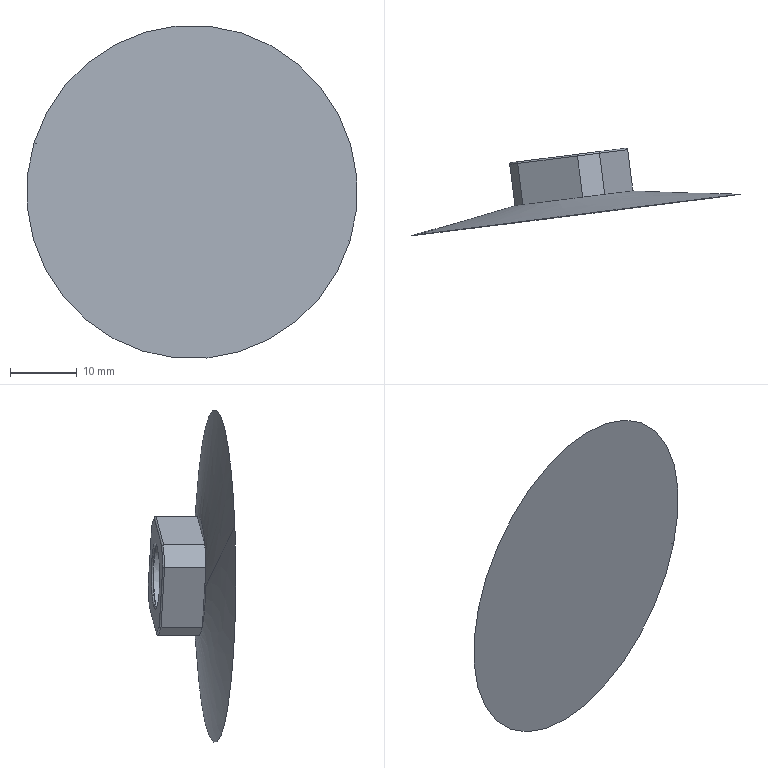Component | SolidWorks | SuctionCup-1 | 1 solid | 35 faces | box 49.61 x 13.13 x 50 mm | volume 3362 mm3 | plane 19 | cylinder 8 | torus 4 | spline 2 | sphere 2 | commonest cylinder face diameters 0.5 x8
STEP:
#1=COLOUR_RGB('',0.7922,0.8196,0.9333);
#2=FILL_AREA_STYLE_COLOUR('',#1);
#3=FILL_AREA_STYLE('',(#2));
#4=SURFACE_STYLE_FILL_AREA(#3);
#5=SURFACE_SIDE_STYLE('',(#4));
#6=SURFACE_STYLE_USAGE(.BOTH.,#5);
#7=PRESENTATION_STYLE_ASSIGNMENT((#6));
#8=CARTESIAN_POINT('',(20.728,-12.767,5.415));
#9=VERTEX_POINT('',#8);
#10=CARTESIAN_POINT('',(20.728,-12.77,5.415));
#11=VERTEX_POINT('',#10);
#12=CARTESIAN_POINT('',(20.724,-12.767,5.424));
#13=DIRECTION('',(-0.8974,-0.113,-0.4265));
#14=DIRECTION('',(-0.4293,0.,0.9032));
#15=AXIS2_PLACEMENT_3D('',#12,#13,#14);
#16=CIRCLE('',#15,0.009843);
#17=EDGE_CURVE('',#9,#11,#16,.T.);
#18=ORIENTED_EDGE('',*,*,#17,.F.);
#19=CARTESIAN_POINT('',(20.887,-12.747,5.074));
#20=VERTEX_POINT('',#19);
#21=CARTESIAN_POINT('',(20.808,-12.757,5.245));
#22=DIRECTION('',(-0.1249,0.9922,-0.));
#23=DIRECTION('',(-0.9922,-0.1249,0.));
#24=AXIS2_PLACEMENT_3D('',#21,#22,#23);
#25=CIRCLE('',#24,0.1882);
#26=EDGE_CURVE('',#9,#20,#25,.T.);
#27=ORIENTED_EDGE('',*,*,#26,.T.);
#28=CARTESIAN_POINT('',(20.888,-12.75,5.074));
#29=VERTEX_POINT('',#28);
#30=CARTESIAN_POINT('',(20.891,-12.746,5.065));
#31=DIRECTION('',(0.8974,0.113,0.4265));
#32=DIRECTION('',(0.4293,0.,-0.9032));
#33=AXIS2_PLACEMENT_3D('',#30,#31,#32);
#34=CIRCLE('',#33,0.009843);
#35=EDGE_CURVE('',#20,#29,#34,.T.);
#36=ORIENTED_EDGE('',*,*,#35,.T.);
#37=CARTESIAN_POINT('',(20.808,-12.76,5.245));
#38=DIRECTION('',(-0.1249,0.9922,-0.));
#39=DIRECTION('',(-0.4232,-0.05327,0.9045));
#40=AXIS2_PLACEMENT_3D('',#37,#38,#39);
#41=CIRCLE('',#40,0.1886);
#42=EDGE_CURVE('',#11,#29,#41,.T.);
#43=ORIENTED_EDGE('',*,*,#42,.F.);
#44=EDGE_LOOP('',(#18,#27,#36,#43));
#45=FACE_OUTER_BOUND('',#44,.T.);
#46=CARTESIAN_POINT('',(20.808,-12.757,5.245));
#47=DIRECTION('',(-0.1249,0.9922,-0.));
#48=DIRECTION('',(0.4232,0.05327,-0.9045));
#49=AXIS2_PLACEMENT_3D('',#46,#47,#48);
#50=TOROIDAL_SURFACE('',#49,0.1981,0.009843);
#51=ADVANCED_FACE('',(#45),#50,.T.);
#52=ORIENTED_EDGE('',*,*,#35,.F.);
#53=CARTESIAN_POINT('',(20.808,-12.757,5.245));
#54=DIRECTION('',(-0.1249,0.9922,-0.));
#55=DIRECTION('',(-0.9922,-0.1249,0.));
#56=AXIS2_PLACEMENT_3D('',#53,#54,#55);
#57=CIRCLE('',#56,0.1882);
#58=EDGE_CURVE('',#20,#9,#57,.T.);
#59=ORIENTED_EDGE('',*,*,#58,.T.);
#60=ORIENTED_EDGE('',*,*,#17,.T.);
#61=CARTESIAN_POINT('',(20.808,-12.76,5.245));
#62=DIRECTION('',(-0.1249,0.9922,-0.));
#63=DIRECTION('',(-0.4232,-0.05327,0.9045));
#64=AXIS2_PLACEMENT_3D('',#61,#62,#63);
#65=CIRCLE('',#64,0.1886);
#66=EDGE_CURVE('',#29,#11,#65,.T.);
#67=ORIENTED_EDGE('',*,*,#66,.F.);
#68=EDGE_LOOP('',(#52,#59,#60,#67));
#69=FACE_OUTER_BOUND('',#68,.T.);
#70=CARTESIAN_POINT('',(20.808,-12.757,5.245));
#71=DIRECTION('',(-0.1249,0.9922,-0.));
#72=DIRECTION('',(0.4232,0.05327,-0.9045));
#73=AXIS2_PLACEMENT_3D('',#70,#71,#72);
#74=TOROIDAL_SURFACE('',#73,0.1981,0.009843);
#75=ADVANCED_FACE('',(#69),#74,.T.);
#76=CARTESIAN_POINT('',(21.187,-12.957,5.192));
#77=VERTEX_POINT('',#76);
#78=CARTESIAN_POINT('',(21.185,-12.957,5.304));
#79=VERTEX_POINT('',#78);
#80=CARTESIAN_POINT('',(20.838,-13.001,5.245));
#81=DIRECTION('',(0.1249,-0.9922,0.));
#82=DIRECTION('',(-0.4232,-0.05327,0.9045));
#83=AXIS2_PLACEMENT_3D('',#80,#81,#82);
#84=CIRCLE('',#83,0.3549);
#85=EDGE_CURVE('',#77,#79,#84,.T.);
#86=ORIENTED_EDGE('',*,*,#85,.T.);
#87=CARTESIAN_POINT('',(21.783,-12.981,4.952));
#88=VERTEX_POINT('',#87);
#89=CARTESIAN_POINT('',(21.185,-12.957,5.304));
#90=CARTESIAN_POINT('',(21.783,-12.981,4.952));
#91=B_SPLINE_CURVE_WITH_KNOTS('',1,(#89,#90),.UNSPECIFIED.,.F.,.F.,(2,2),(0.,1.),.UNSPECIFIED.);
#92=EDGE_CURVE('',#79,#88,#91,.T.);
#93=ORIENTED_EDGE('',*,*,#92,.T.);
#94=CARTESIAN_POINT('',(19.918,-13.216,5.537));
#95=VERTEX_POINT('',#94);
#96=CARTESIAN_POINT('',(20.851,-13.099,5.245));
#97=DIRECTION('',(0.1249,-0.9922,0.));
#98=DIRECTION('',(-0.4232,-0.05327,0.9045));
#99=AXIS2_PLACEMENT_3D('',#96,#97,#98);
#100=CIRCLE('',#99,0.9843);
#101=EDGE_CURVE('',#95,#88,#100,.T.);
#102=ORIENTED_EDGE('',*,*,#101,.F.);
#103=CARTESIAN_POINT('',(20.491,-13.045,5.185));
#104=VERTEX_POINT('',#103);
#105=CARTESIAN_POINT('',(20.491,-13.045,5.185));
#106=CARTESIAN_POINT('',(19.918,-13.216,5.537));
#107=B_SPLINE_CURVE_WITH_KNOTS('',1,(#105,#106),.UNSPECIFIED.,.F.,.F.,(2,2),(0.,1.),.UNSPECIFIED.);
#108=EDGE_CURVE('',#104,#95,#107,.T.);
#109=ORIENTED_EDGE('',*,*,#108,.F.);
#110=CARTESIAN_POINT('',(20.657,-13.024,4.941));
#111=VERTEX_POINT('',#110);
#112=CARTESIAN_POINT('',(20.838,-13.001,5.245));
#113=DIRECTION('',(0.1249,-0.9922,0.));
#114=DIRECTION('',(-0.4232,-0.05327,0.9045));
#115=AXIS2_PLACEMENT_3D('',#112,#113,#114);
#116=CIRCLE('',#115,0.3549);
#117=EDGE_CURVE('',#104,#111,#116,.T.);
#118=ORIENTED_EDGE('',*,*,#117,.T.);
#119=CARTESIAN_POINT('',(20.787,-13.007,4.894));
#120=VERTEX_POINT('',#119);
#121=CARTESIAN_POINT('',(20.838,-13.001,5.245));
#122=DIRECTION('',(0.1249,-0.9922,0.));
#123=DIRECTION('',(-0.4232,-0.05327,0.9045));
#124=AXIS2_PLACEMENT_3D('',#121,#122,#123);
#125=CIRCLE('',#124,0.3549);
#126=EDGE_CURVE('',#111,#120,#125,.T.);
#127=ORIENTED_EDGE('',*,*,#126,.T.);
#128=CARTESIAN_POINT('',(21.14,-12.963,5.061));
#129=VERTEX_POINT('',#128);
#130=CARTESIAN_POINT('',(20.838,-13.001,5.245));
#131=DIRECTION('',(0.1249,-0.9922,0.));
#132=DIRECTION('',(-0.4232,-0.05327,0.9045));
#133=AXIS2_PLACEMENT_3D('',#130,#131,#132);
#134=CIRCLE('',#133,0.3549);
#135=EDGE_CURVE('',#120,#129,#134,.T.);
#136=ORIENTED_EDGE('',*,*,#135,.T.);
#137=CARTESIAN_POINT('',(20.838,-13.001,5.245));
#138=DIRECTION('',(0.1249,-0.9922,0.));
#139=DIRECTION('',(-0.4232,-0.05327,0.9045));
#140=AXIS2_PLACEMENT_3D('',#137,#138,#139);
#141=CIRCLE('',#140,0.3549);
#142=EDGE_CURVE('',#129,#77,#141,.T.);
#143=ORIENTED_EDGE('',*,*,#142,.T.);
#144=EDGE_LOOP('',(#86,#93,#102,#109,#118,#127,#136,#143));
#145=FACE_OUTER_BOUND('',#144,.T.);
#146=CARTESIAN_POINT('',(20.491,-13.045,5.185));
#147=CARTESIAN_POINT('',(19.918,-13.216,5.537));
#148=CARTESIAN_POINT('',(20.609,-13.03,4.485));
#149=CARTESIAN_POINT('',(19.337,-13.289,3.658));
#150=CARTESIAN_POINT('',(21.303,-12.942,4.604));
#151=CARTESIAN_POINT('',(21.202,-13.054,3.072));
#152=CARTESIAN_POINT('',(21.185,-12.957,5.304));
#153=CARTESIAN_POINT('',(21.783,-12.981,4.952));
#154=CARTESIAN_POINT('',(21.068,-12.972,6.004));
#155=CARTESIAN_POINT('',(22.364,-12.908,6.831));
#156=CARTESIAN_POINT('',(20.373,-13.059,5.885));
#157=CARTESIAN_POINT('',(20.499,-13.143,7.417));
#158=CARTESIAN_POINT('',(20.491,-13.045,5.185));
#159=CARTESIAN_POINT('',(19.918,-13.216,5.537));
#160=(BOUNDED_SURFACE()B_SPLINE_SURFACE(3,1,((#146,#147),(#148,#149),(#150,#151),(#152,#153),(#154,#155),(#156,#157),(#158,#159)),.UNSPECIFIED.,.T.,.F.,.F.)B_SPLINE_SURFACE_WITH_KNOTS((4,3,4),(2,2),(0.,0.5,1.),(0.,1.),.UNSPECIFIED.)GEOMETRIC_REPRESENTATION_ITEM()RATIONAL_B_SPLINE_SURFACE(((1.,1.),(0.3333,0.3333),(0.3333,0.3333),(1.,1.),(0.3333,0.3333),(0.3333,0.3333),(1.,1.)))REPRESENTATION_ITEM('')SURFACE());
#161=ADVANCED_FACE('',(#145),#160,.T.);
#162=ORIENTED_EDGE('',*,*,#58,.F.);
#163=CARTESIAN_POINT('',(20.89,-12.737,5.065));
#164=VERTEX_POINT('',#163);
#165=CARTESIAN_POINT('',(20.891,-12.746,5.065));
#166=DIRECTION('',(0.8974,0.113,0.4265));
#167=DIRECTION('',(0.4293,0.,-0.9032));
#168=AXIS2_PLACEMENT_3D('',#165,#166,#167);
#169=CIRCLE('',#168,0.009843);
#170=EDGE_CURVE('',#164,#20,#169,.T.);
#171=ORIENTED_EDGE('',*,*,#170,.F.);
#172=CARTESIAN_POINT('',(20.722,-12.758,5.424));
#173=VERTEX_POINT('',#172);
#174=CARTESIAN_POINT('',(20.806,-12.747,5.245));
#175=DIRECTION('',(0.1249,-0.9922,0.));
#176=DIRECTION('',(0.4232,0.05327,-0.9045));
#177=AXIS2_PLACEMENT_3D('',#174,#175,#176);
#178=CIRCLE('',#177,0.1981);
#179=EDGE_CURVE('',#173,#164,#178,.T.);
#180=ORIENTED_EDGE('',*,*,#179,.F.);
#181=CARTESIAN_POINT('',(20.724,-12.767,5.424));
#182=DIRECTION('',(-0.8974,-0.113,-0.4265));
#183=DIRECTION('',(-0.4293,0.,0.9032));
#184=AXIS2_PLACEMENT_3D('',#181,#182,#183);
#185=CIRCLE('',#184,0.009843);
#186=EDGE_CURVE('',#173,#9,#185,.T.);
#187=ORIENTED_EDGE('',*,*,#186,.T.);
#188=EDGE_LOOP('',(#162,#171,#180,#187));
#189=FACE_OUTER_BOUND('',#188,.T.);
#190=CARTESIAN_POINT('',(20.808,-12.757,5.245));
#191=DIRECTION('',(-0.1249,0.9922,-0.));
#192=DIRECTION('',(0.4232,0.05327,-0.9045));
#193=AXIS2_PLACEMENT_3D('',#190,#191,#192);
#194=TOROIDAL_SURFACE('',#193,0.1981,0.009843);
#195=ADVANCED_FACE('',(#189),#194,.T.);
#196=CARTESIAN_POINT('',(20.864,-12.998,5.189));
#197=VERTEX_POINT('',#196);
#198=CARTESIAN_POINT('',(20.812,-13.004,5.3));
#199=VERTEX_POINT('',#198);
#200=CARTESIAN_POINT('',(20.838,-13.001,5.245));
#201=DIRECTION('',(-0.1249,0.9922,-0.));
#202=DIRECTION('',(0.4232,0.05327,-0.9045));
#203=AXIS2_PLACEMENT_3D('',#200,#201,#202);
#204=CIRCLE('',#203,0.06147);
#205=EDGE_CURVE('',#197,#199,#204,.T.);
#206=ORIENTED_EDGE('',*,*,#205,.F.);
#207=CARTESIAN_POINT('',(20.815,-12.815,5.245));
#208=DIRECTION('',(0.8974,0.113,0.4265));
#209=DIRECTION('',(0.4293,0.,-0.9032));
#210=AXIS2_PLACEMENT_3D('',#207,#208,#209);
#211=CIRCLE('',#210,0.1969);
#212=EDGE_CURVE('',#197,#29,#211,.T.);
#213=ORIENTED_EDGE('',*,*,#212,.T.);
#214=ORIENTED_EDGE('',*,*,#66,.T.);
#215=CARTESIAN_POINT('',(20.815,-12.815,5.245));
#216=DIRECTION('',(-0.8974,-0.113,-0.4265));
#217=DIRECTION('',(-0.4293,0.,0.9032));
#218=AXIS2_PLACEMENT_3D('',#215,#216,#217);
#219=CIRCLE('',#218,0.1969);
#220=EDGE_CURVE('',#199,#11,#219,.T.);
#221=ORIENTED_EDGE('',*,*,#220,.F.);
#222=EDGE_LOOP('',(#206,#213,#214,#221));
#223=FACE_OUTER_BOUND('',#222,.T.);
#224=CARTESIAN_POINT('',(20.815,-12.815,5.245));
#225=DIRECTION('',(0.8974,0.113,0.4265));
#226=DIRECTION('',(-0.4232,-0.05327,0.9045));
#227=AXIS2_PLACEMENT_3D('',#224,#225,#226);
#228=SPHERICAL_SURFACE('',#227,0.1969);
#229=ADVANCED_FACE('',(#223),#228,.F.);
#230=CARTESIAN_POINT('',(20.89,-12.994,5.596));
#231=VERTEX_POINT('',#230);
#232=CARTESIAN_POINT('',(20.859,-12.75,5.596));
#233=VERTEX_POINT('',#232);
#234=CARTESIAN_POINT('',(20.89,-12.994,5.596));
#235=DIRECTION('',(-0.1249,0.9922,-0.));
#236=VECTOR('',#235,39.37);
#237=LINE('',#234,#236);
#238=EDGE_CURVE('',#231,#233,#237,.T.);
#239=ORIENTED_EDGE('',*,*,#238,.T.);
#240=CARTESIAN_POINT('',(20.506,-12.795,5.428));
#241=VERTEX_POINT('',#240);
#242=CARTESIAN_POINT('',(20.506,-12.795,5.428));
#243=DIRECTION('',(-0.8974,-0.113,-0.4265));
#244=VECTOR('',#243,39.37);
#245=LINE('',#242,#244);
#246=EDGE_CURVE('',#233,#241,#245,.T.);
#247=ORIENTED_EDGE('',*,*,#246,.T.);
#248=CARTESIAN_POINT('',(20.537,-13.039,5.428));
#249=VERTEX_POINT('',#248);
#250=CARTESIAN_POINT('',(20.537,-13.039,5.428));
#251=DIRECTION('',(0.1249,-0.9922,0.));
#252=VECTOR('',#251,39.37);
#253=LINE('',#250,#252);
#254=EDGE_CURVE('',#241,#249,#253,.T.);
#255=ORIENTED_EDGE('',*,*,#254,.T.);
#256=CARTESIAN_POINT('',(20.978,-12.983,5.638));
#257=DIRECTION('',(-0.8974,-0.113,-0.4265));
#258=VECTOR('',#257,39.37);
#259=LINE('',#256,#258);
#260=EDGE_CURVE('',#231,#249,#259,.T.);
#261=ORIENTED_EDGE('',*,*,#260,.F.);
#262=EDGE_LOOP('',(#239,#247,#255,#261));
#263=FACE_OUTER_BOUND('',#262,.T.);
#264=CARTESIAN_POINT('',(20.978,-12.983,5.638));
#265=DIRECTION('',(0.4232,0.05327,-0.9045));
#266=DIRECTION('',(0.1249,-0.9922,0.));
#267=AXIS2_PLACEMENT_3D('',#264,#265,#266);
#268=PLANE('',#267);
#269=ADVANCED_FACE('',(#263),#268,.F.);
#270=CARTESIAN_POINT('',(20.49,-13.045,5.297));
#271=VERTEX_POINT('',#270);
#272=CARTESIAN_POINT('',(20.459,-12.801,5.297));
#273=VERTEX_POINT('',#272);
#274=CARTESIAN_POINT('',(20.49,-13.045,5.297));
#275=DIRECTION('',(-0.1249,0.9922,-0.));
#276=VECTOR('',#275,39.37);
#277=LINE('',#274,#276);
#278=EDGE_CURVE('',#271,#273,#277,.T.);
#279=ORIENTED_EDGE('',*,*,#278,.T.);
#280=CARTESIAN_POINT('',(20.626,-12.78,4.941));
#281=VERTEX_POINT('',#280);
#282=CARTESIAN_POINT('',(20.626,-12.78,4.941));
#283=DIRECTION('',(0.4232,0.05327,-0.9045));
#284=VECTOR('',#283,39.37);
#285=LINE('',#282,#284);
#286=EDGE_CURVE('',#273,#281,#285,.T.);
#287=ORIENTED_EDGE('',*,*,#286,.T.);
#288=CARTESIAN_POINT('',(20.657,-13.024,4.941));
#289=DIRECTION('',(0.1249,-0.9922,0.));
#290=VECTOR('',#289,39.37);
#291=LINE('',#288,#290);
#292=EDGE_CURVE('',#281,#111,#291,.T.);
#293=ORIENTED_EDGE('',*,*,#292,.T.);
#294=CARTESIAN_POINT('',(20.698,-13.019,4.852));
#295=DIRECTION('',(0.4232,0.05327,-0.9045));
#296=VECTOR('',#295,39.37);
#297=LINE('',#294,#296);
#298=EDGE_CURVE('',#271,#111,#297,.T.);
#299=ORIENTED_EDGE('',*,*,#298,.F.);
#300=EDGE_LOOP('',(#279,#287,#293,#299));
#301=FACE_OUTER_BOUND('',#300,.T.);
#302=CARTESIAN_POINT('',(20.698,-13.019,4.852));
#303=DIRECTION('',(0.8974,0.113,0.4265));
#304=DIRECTION('',(-0.1249,0.9922,-0.));
#305=AXIS2_PLACEMENT_3D('',#302,#303,#304);
#306=PLANE('',#305);
#307=ADVANCED_FACE('',(#301),#306,.F.);
#308=CARTESIAN_POINT('',(20.756,-12.763,4.894));
#309=VERTEX_POINT('',#308);
#310=CARTESIAN_POINT('',(20.787,-13.007,4.894));
#311=DIRECTION('',(-0.1249,0.9922,-0.));
#312=VECTOR('',#311,39.37);
#313=LINE('',#310,#312);
#314=EDGE_CURVE('',#120,#309,#313,.T.);
#315=ORIENTED_EDGE('',*,*,#314,.T.);
#316=CARTESIAN_POINT('',(21.109,-12.719,5.061));
#317=VERTEX_POINT('',#316);
#318=CARTESIAN_POINT('',(21.109,-12.719,5.061));
#319=DIRECTION('',(0.8974,0.113,0.4265));
#320=VECTOR('',#319,39.37);
#321=LINE('',#318,#320);
#322=EDGE_CURVE('',#309,#317,#321,.T.);
#323=ORIENTED_EDGE('',*,*,#322,.T.);
#324=CARTESIAN_POINT('',(21.14,-12.963,5.061));
#325=DIRECTION('',(0.1249,-0.9922,0.));
#326=VECTOR('',#325,39.37);
#327=LINE('',#324,#326);
#328=EDGE_CURVE('',#317,#129,#327,.T.);
#329=ORIENTED_EDGE('',*,*,#328,.T.);
#330=CARTESIAN_POINT('',(21.228,-12.952,5.103));
#331=DIRECTION('',(0.8974,0.113,0.4265));
#332=VECTOR('',#331,39.37);
#333=LINE('',#330,#332);
#334=EDGE_CURVE('',#120,#129,#333,.T.);
#335=ORIENTED_EDGE('',*,*,#334,.F.);
#336=EDGE_LOOP('',(#315,#323,#329,#335));
#337=FACE_OUTER_BOUND('',#336,.T.);
#338=CARTESIAN_POINT('',(21.228,-12.952,5.103));
#339=DIRECTION('',(-0.4232,-0.05327,0.9045));
#340=DIRECTION('',(-0.1249,0.9922,-0.));
#341=AXIS2_PLACEMENT_3D('',#338,#339,#340);
#342=PLANE('',#341);
#343=ADVANCED_FACE('',(#337),#342,.F.);
#344=CARTESIAN_POINT('',(21.156,-12.713,5.192));
#345=VERTEX_POINT('',#344);
#346=CARTESIAN_POINT('',(21.187,-12.957,5.192));
#347=DIRECTION('',(-0.1249,0.9922,-0.));
#348=VECTOR('',#347,39.37);
#349=LINE('',#346,#348);
#350=EDGE_CURVE('',#77,#345,#349,.T.);
#351=ORIENTED_EDGE('',*,*,#350,.T.);
#352=CARTESIAN_POINT('',(20.989,-12.734,5.549));
#353=VERTEX_POINT('',#352);
#354=CARTESIAN_POINT('',(20.989,-12.734,5.549));
#355=DIRECTION('',(-0.4232,-0.05327,0.9045));
#356=VECTOR('',#355,39.37);
#357=LINE('',#354,#356);
#358=EDGE_CURVE('',#345,#353,#357,.T.);
#359=ORIENTED_EDGE('',*,*,#358,.T.);
#360=CARTESIAN_POINT('',(21.02,-12.978,5.549));
#361=VERTEX_POINT('',#360);
#362=CARTESIAN_POINT('',(21.02,-12.978,5.549));
#363=DIRECTION('',(0.1249,-0.9922,0.));
#364=VECTOR('',#363,39.37);
#365=LINE('',#362,#364);
#366=EDGE_CURVE('',#353,#361,#365,.T.);
#367=ORIENTED_EDGE('',*,*,#366,.T.);
#368=CARTESIAN_POINT('',(21.228,-12.952,5.103));
#369=DIRECTION('',(-0.4232,-0.05327,0.9045));
#370=VECTOR('',#369,39.37);
#371=LINE('',#368,#370);
#372=EDGE_CURVE('',#77,#361,#371,.T.);
#373=ORIENTED_EDGE('',*,*,#372,.F.);
#374=EDGE_LOOP('',(#351,#359,#367,#373));
#375=FACE_OUTER_BOUND('',#374,.T.);
#376=CARTESIAN_POINT('',(21.228,-12.952,5.103));
#377=DIRECTION('',(-0.8974,-0.113,-0.4265));
#378=DIRECTION('',(0.1249,-0.9922,0.));
#379=AXIS2_PLACEMENT_3D('',#376,#377,#378);
#380=PLANE('',#379);
#381=ADVANCED_FACE('',(#375),#380,.F.);
#382=CARTESIAN_POINT('',(20.632,-12.769,4.948));
#383=VERTEX_POINT('',#382);
#384=CARTESIAN_POINT('',(20.469,-12.79,5.297));
#385=VERTEX_POINT('',#384);
#386=CARTESIAN_POINT('',(20.467,-12.79,5.301));
#387=DIRECTION('',(-0.4232,-0.05327,0.9045));
#388=VECTOR('',#387,39.37);
#389=LINE('',#386,#388);
#390=EDGE_CURVE('',#383,#385,#389,.T.);
#391=ORIENTED_EDGE('',*,*,#390,.T.);
#392=CARTESIAN_POINT('',(20.513,-12.784,5.421));
#393=VERTEX_POINT('',#392);
#394=CARTESIAN_POINT('',(20.491,-12.787,5.359));
#395=DIRECTION('',(0.3353,0.04221,0.9412));
#396=VECTOR('',#395,39.37);
#397=LINE('',#394,#396);
#398=EDGE_CURVE('',#385,#393,#397,.T.);
#399=ORIENTED_EDGE('',*,*,#398,.T.);
#400=CARTESIAN_POINT('',(20.859,-12.741,5.585));
#401=VERTEX_POINT('',#400);
#402=CARTESIAN_POINT('',(20.862,-12.74,5.587));
#403=DIRECTION('',(0.8974,0.113,0.4265));
#404=VECTOR('',#403,39.37);
#405=LINE('',#402,#404);
#406=EDGE_CURVE('',#393,#401,#405,.T.);
#407=ORIENTED_EDGE('',*,*,#406,.T.);
#408=CARTESIAN_POINT('',(20.981,-12.725,5.541));
#409=VERTEX_POINT('',#408);
#410=CARTESIAN_POINT('',(20.92,-12.733,5.563));
#411=DIRECTION('',(0.9338,0.1175,-0.338));
#412=VECTOR('',#411,39.37);
#413=LINE('',#410,#412);
#414=EDGE_CURVE('',#401,#409,#413,.T.);
#415=ORIENTED_EDGE('',*,*,#414,.T.);
#416=CARTESIAN_POINT('',(21.144,-12.705,5.192));
#417=VERTEX_POINT('',#416);
#418=CARTESIAN_POINT('',(21.146,-12.704,5.188));
#419=DIRECTION('',(0.4232,0.05327,-0.9045));
#420=VECTOR('',#419,39.37);
#421=LINE('',#418,#420);
#422=EDGE_CURVE('',#409,#417,#421,.T.);
#423=ORIENTED_EDGE('',*,*,#422,.T.);
#424=CARTESIAN_POINT('',(21.1,-12.71,5.069));
#425=VERTEX_POINT('',#424);
#426=CARTESIAN_POINT('',(21.122,-12.707,5.13));
#427=DIRECTION('',(-0.3353,-0.04221,-0.9412));
#428=VECTOR('',#427,39.37);
#429=LINE('',#426,#428);
#430=EDGE_CURVE('',#417,#425,#429,.T.);
#431=ORIENTED_EDGE('',*,*,#430,.T.);
#432=CARTESIAN_POINT('',(20.754,-12.754,4.904));
#433=VERTEX_POINT('',#432);
#434=CARTESIAN_POINT('',(20.75,-12.754,4.902));
#435=DIRECTION('',(-0.8974,-0.113,-0.4265));
#436=VECTOR('',#435,39.37);
#437=LINE('',#434,#436);
#438=EDGE_CURVE('',#425,#433,#437,.T.);
#439=ORIENTED_EDGE('',*,*,#438,.T.);
#440=CARTESIAN_POINT('',(20.693,-12.761,4.926));
#441=DIRECTION('',(-0.9338,-0.1175,0.338));
#442=VECTOR('',#441,39.37);
#443=LINE('',#440,#442);
#444=EDGE_CURVE('',#433,#383,#443,.T.);
#445=ORIENTED_EDGE('',*,*,#444,.T.);
#446=EDGE_LOOP('',(#391,#399,#407,#415,#423,#431,#439,#445));
#447=FACE_OUTER_BOUND('',#446,.T.);
#448=CARTESIAN_POINT('',(20.806,-12.747,5.245));
#449=DIRECTION('',(0.1249,-0.9922,0.));
#450=DIRECTION('',(0.4232,0.05327,-0.9045));
#451=AXIS2_PLACEMENT_3D('',#448,#449,#450);
#452=CIRCLE('',#451,0.1981);
#453=EDGE_CURVE('',#164,#173,#452,.T.);
#454=ORIENTED_EDGE('',*,*,#453,.T.);
#455=ORIENTED_EDGE('',*,*,#179,.T.);
#456=EDGE_LOOP('',(#454,#455));
#457=FACE_BOUND('',#456,.T.);
#458=CARTESIAN_POINT('',(20.806,-12.747,5.245));
#459=DIRECTION('',(-0.1249,0.9922,-0.));
#460=DIRECTION('',(0.4232,0.05327,-0.9045));
#461=AXIS2_PLACEMENT_3D('',#458,#459,#460);
#462=PLANE('',#461);
#463=ADVANCED_FACE('',(#447,#457),#462,.T.);
#464=ORIENTED_EDGE('',*,*,#366,.F.);
#465=CARTESIAN_POINT('',(20.859,-12.75,5.596));
#466=DIRECTION('',(-0.9338,-0.1175,0.338));
#467=VECTOR('',#466,39.37);
#468=LINE('',#465,#467);
#469=EDGE_CURVE('',#353,#233,#468,.T.);
#470=ORIENTED_EDGE('',*,*,#469,.T.);
#471=ORIENTED_EDGE('',*,*,#238,.F.);
#472=CARTESIAN_POINT('',(20.89,-12.994,5.596));
#473=DIRECTION('',(-0.9338,-0.1175,0.338));
#474=VECTOR('',#473,39.37);
#475=LINE('',#472,#474);
#476=EDGE_CURVE('',#361,#231,#475,.T.);
#477=ORIENTED_EDGE('',*,*,#476,.F.);
#478=EDGE_LOOP('',(#464,#470,#471,#477));
#479=FACE_OUTER_BOUND('',#478,.T.);
#480=CARTESIAN_POINT('',(20.89,-12.994,5.596));
#481=DIRECTION('',(-0.3353,-0.04221,-0.9412));
#482=DIRECTION('',(-0.1249,0.9922,-0.));
#483=AXIS2_PLACEMENT_3D('',#480,#481,#482);
#484=PLANE('',#483);
#485=ADVANCED_FACE('',(#479),#484,.F.);
#486=ORIENTED_EDGE('',*,*,#328,.F.);
#487=CARTESIAN_POINT('',(21.156,-12.713,5.192));
#488=DIRECTION('',(0.3353,0.04221,0.9412));
#489=VECTOR('',#488,39.37);
#490=LINE('',#487,#489);
#491=EDGE_CURVE('',#317,#345,#490,.T.);
#492=ORIENTED_EDGE('',*,*,#491,.T.);
#493=ORIENTED_EDGE('',*,*,#350,.F.);
#494=CARTESIAN_POINT('',(21.187,-12.957,5.192));
#495=DIRECTION('',(0.3353,0.04221,0.9412));
#496=VECTOR('',#495,39.37);
#497=LINE('',#494,#496);
#498=EDGE_CURVE('',#129,#77,#497,.T.);
#499=ORIENTED_EDGE('',*,*,#498,.F.);
#500=EDGE_LOOP('',(#486,#492,#493,#499));
#501=FACE_OUTER_BOUND('',#500,.T.);
#502=CARTESIAN_POINT('',(21.187,-12.957,5.192));
#503=DIRECTION('',(-0.9338,-0.1175,0.338));
#504=DIRECTION('',(-0.1249,0.9922,-0.));
#505=AXIS2_PLACEMENT_3D('',#502,#503,#504);
#506=PLANE('',#505);
#507=ADVANCED_FACE('',(#501),#506,.F.);
#508=ORIENTED_EDGE('',*,*,#292,.F.);
#509=CARTESIAN_POINT('',(20.756,-12.763,4.894));
#510=DIRECTION('',(0.9338,0.1175,-0.338));
#511=VECTOR('',#510,39.37);
#512=LINE('',#509,#511);
#513=EDGE_CURVE('',#281,#309,#512,.T.);
#514=ORIENTED_EDGE('',*,*,#513,.T.);
#515=ORIENTED_EDGE('',*,*,#314,.F.);
#516=CARTESIAN_POINT('',(20.787,-13.007,4.894));
#517=DIRECTION('',(0.9338,0.1175,-0.338));
#518=VECTOR('',#517,39.37);
#519=LINE('',#516,#518);
#520=EDGE_CURVE('',#111,#120,#519,.T.);
#521=ORIENTED_EDGE('',*,*,#520,.F.);
#522=EDGE_LOOP('',(#508,#514,#515,#521));
#523=FACE_OUTER_BOUND('',#522,.T.);
#524=CARTESIAN_POINT('',(20.787,-13.007,4.894));
#525=DIRECTION('',(0.3353,0.04221,0.9412));
#526=DIRECTION('',(-0.1249,0.9922,-0.));
#527=AXIS2_PLACEMENT_3D('',#524,#525,#526);
#528=PLANE('',#527);
#529=ADVANCED_FACE('',(#523),#528,.F.);
#530=ORIENTED_EDGE('',*,*,#254,.F.);
#531=CARTESIAN_POINT('',(20.459,-12.801,5.297));
#532=DIRECTION('',(-0.3353,-0.04221,-0.9412));
#533=VECTOR('',#532,39.37);
#534=LINE('',#531,#533);
#535=EDGE_CURVE('',#241,#273,#534,.T.);
#536=ORIENTED_EDGE('',*,*,#535,.T.);
#537=ORIENTED_EDGE('',*,*,#278,.F.);
#538=CARTESIAN_POINT('',(20.49,-13.045,5.297));
#539=DIRECTION('',(-0.3353,-0.04221,-0.9412));
#540=VECTOR('',#539,39.37);
#541=LINE('',#538,#540);
#542=EDGE_CURVE('',#249,#271,#541,.T.);
#543=ORIENTED_EDGE('',*,*,#542,.F.);
#544=EDGE_LOOP('',(#530,#536,#537,#543));
#545=FACE_OUTER_BOUND('',#544,.T.);
#546=CARTESIAN_POINT('',(20.49,-13.045,5.297));
#547=DIRECTION('',(0.9338,0.1175,-0.338));
#548=DIRECTION('',(-0.1249,0.9922,-0.));
#549=AXIS2_PLACEMENT_3D('',#546,#547,#548);
#550=PLANE('',#549);
#551=ADVANCED_FACE('',(#545),#550,.F.);
#552=ORIENTED_EDGE('',*,*,#212,.F.);
#553=CARTESIAN_POINT('',(20.838,-13.001,5.245));
#554=DIRECTION('',(-0.1249,0.9922,-0.));
#555=DIRECTION('',(0.4232,0.05327,-0.9045));
#556=AXIS2_PLACEMENT_3D('',#553,#554,#555);
#557=CIRCLE('',#556,0.06147);
#558=EDGE_CURVE('',#199,#197,#557,.T.);
#559=ORIENTED_EDGE('',*,*,#558,.F.);
#560=ORIENTED_EDGE('',*,*,#220,.T.);
#561=ORIENTED_EDGE('',*,*,#42,.T.);
#562=EDGE_LOOP('',(#552,#559,#560,#561));
#563=FACE_OUTER_BOUND('',#562,.T.);
#564=CARTESIAN_POINT('',(20.815,-12.815,5.245));
#565=DIRECTION('',(0.8974,0.113,0.4265));
#566=DIRECTION('',(-0.4232,-0.05327,0.9045));
#567=AXIS2_PLACEMENT_3D('',#564,#565,#566);
#568=SPHERICAL_SURFACE('',#567,0.1969);
#569=ADVANCED_FACE('',(#563),#568,.F.);
#570=CARTESIAN_POINT('',(21.156,-12.713,5.192));
#571=CARTESIAN_POINT('',(21.155,-12.707,5.192));
#572=CARTESIAN_POINT('',(21.15,-12.704,5.192));
#573=CARTESIAN_POINT('',(21.144,-12.705,5.192));
#574=(BOUNDED_CURVE()B_SPLINE_CURVE(3,(#570,#571,#572,#573),.UNSPECIFIED.,.F.,.F.)B_SPLINE_CURVE_WITH_KNOTS((4,4),(0.,1.571),.UNSPECIFIED.)CURVE()GEOMETRIC_REPRESENTATION_ITEM()RATIONAL_B_SPLINE_CURVE((1.,0.8047,0.8047,1.))REPRESENTATION_ITEM(''));
#575=EDGE_CURVE('',#345,#417,#574,.T.);
#576=ORIENTED_EDGE('',*,*,#575,.F.);
#577=ORIENTED_EDGE('',*,*,#491,.F.);
#578=CARTESIAN_POINT('',(21.1,-12.71,5.069));
#579=CARTESIAN_POINT('',(21.105,-12.71,5.064));
#580=CARTESIAN_POINT('',(21.108,-12.713,5.061));
#581=CARTESIAN_POINT('',(21.109,-12.719,5.061));
#582=(BOUNDED_CURVE()B_SPLINE_CURVE(3,(#578,#579,#580,#581),.UNSPECIFIED.,.F.,.F.)B_SPLINE_CURVE_WITH_KNOTS((4,4),(1.571,3.142),.UNSPECIFIED.)CURVE()GEOMETRIC_REPRESENTATION_ITEM()RATIONAL_B_SPLINE_CURVE((1.,0.8047,0.8047,1.))REPRESENTATION_ITEM(''));
#583=EDGE_CURVE('',#425,#317,#582,.T.);
#584=ORIENTED_EDGE('',*,*,#583,.F.);
#585=ORIENTED_EDGE('',*,*,#430,.F.);
#586=EDGE_LOOP('',(#576,#577,#584,#585));
#587=FACE_OUTER_BOUND('',#586,.T.);
#588=CARTESIAN_POINT('',(21.123,-12.717,5.13));
#589=DIRECTION('',(0.3353,0.04221,0.9412));
#590=DIRECTION('',(-0.9338,-0.1175,0.338));
#591=AXIS2_PLACEMENT_3D('',#588,#589,#590);
#592=CYLINDRICAL_SURFACE('',#591,0.009843);
#593=ADVANCED_FACE('',(#587),#592,.T.);
#594=ORIENTED_EDGE('',*,*,#583,.T.);
#595=ORIENTED_EDGE('',*,*,#322,.F.);
#596=CARTESIAN_POINT('',(20.754,-12.754,4.904));
#597=CARTESIAN_POINT('',(20.754,-12.754,4.898));
#598=CARTESIAN_POINT('',(20.755,-12.758,4.894));
#599=CARTESIAN_POINT('',(20.756,-12.763,4.894));
#600=(BOUNDED_CURVE()B_SPLINE_CURVE(3,(#596,#597,#598,#599),.UNSPECIFIED.,.F.,.F.)B_SPLINE_CURVE_WITH_KNOTS((4,4),(4.712,6.283),.UNSPECIFIED.)CURVE()GEOMETRIC_REPRESENTATION_ITEM()RATIONAL_B_SPLINE_CURVE((1.,0.8047,0.8047,1.))REPRESENTATION_ITEM(''));
#601=EDGE_CURVE('',#433,#309,#600,.T.);
#602=ORIENTED_EDGE('',*,*,#601,.F.);
#603=ORIENTED_EDGE('',*,*,#438,.F.);
#604=EDGE_LOOP('',(#594,#595,#602,#603));
#605=FACE_OUTER_BOUND('',#604,.T.);
#606=CARTESIAN_POINT('',(21.193,-12.708,5.112));
#607=DIRECTION('',(-0.8974,-0.113,-0.4265));
#608=DIRECTION('',(0.1249,-0.9922,0.));
#609=AXIS2_PLACEMENT_3D('',#606,#607,#608);
#610=CYLINDRICAL_SURFACE('',#609,0.009843);
#611=ADVANCED_FACE('',(#605),#610,.T.);
#612=ORIENTED_EDGE('',*,*,#575,.T.);
#613=ORIENTED_EDGE('',*,*,#422,.F.);
#614=CARTESIAN_POINT('',(20.989,-12.734,5.549));
#615=CARTESIAN_POINT('',(20.988,-12.728,5.549));
#616=CARTESIAN_POINT('',(20.985,-12.725,5.545));
#617=CARTESIAN_POINT('',(20.981,-12.725,5.541));
#618=(BOUNDED_CURVE()B_SPLINE_CURVE(3,(#614,#615,#616,#617),.UNSPECIFIED.,.F.,.F.)B_SPLINE_CURVE_WITH_KNOTS((4,4),(3.142,4.712),.UNSPECIFIED.)CURVE()GEOMETRIC_REPRESENTATION_ITEM()RATIONAL_B_SPLINE_CURVE((1.,0.8047,0.8047,1.))REPRESENTATION_ITEM(''));
#619=EDGE_CURVE('',#353,#409,#618,.T.);
#620=ORIENTED_EDGE('',*,*,#619,.F.);
#621=ORIENTED_EDGE('',*,*,#358,.F.);
#622=EDGE_LOOP('',(#612,#613,#620,#621));
#623=FACE_OUTER_BOUND('',#622,.T.);
#624=CARTESIAN_POINT('',(21.189,-12.709,5.099));
#625=DIRECTION('',(0.4232,0.05327,-0.9045));
#626=DIRECTION('',(0.1249,-0.9922,0.));
#627=AXIS2_PLACEMENT_3D('',#624,#625,#626);
#628=CYLINDRICAL_SURFACE('',#627,0.009843);
#629=ADVANCED_FACE('',(#623),#628,.T.);
#630=ORIENTED_EDGE('',*,*,#601,.T.);
#631=ORIENTED_EDGE('',*,*,#513,.F.);
#632=CARTESIAN_POINT('',(20.632,-12.769,4.948));
#633=CARTESIAN_POINT('',(20.628,-12.77,4.944));
#634=CARTESIAN_POINT('',(20.625,-12.774,4.941));
#635=CARTESIAN_POINT('',(20.626,-12.78,4.941));
#636=(BOUNDED_CURVE()B_SPLINE_CURVE(3,(#632,#633,#634,#635),.UNSPECIFIED.,.F.,.F.)B_SPLINE_CURVE_WITH_KNOTS((4,4),(1.571,3.142),.UNSPECIFIED.)CURVE()GEOMETRIC_REPRESENTATION_ITEM()RATIONAL_B_SPLINE_CURVE((1.,0.8047,0.8047,1.))REPRESENTATION_ITEM(''));
#637=EDGE_CURVE('',#383,#281,#636,.T.);
#638=ORIENTED_EDGE('',*,*,#637,.F.);
#639=ORIENTED_EDGE('',*,*,#444,.F.);
#640=EDGE_LOOP('',(#630,#631,#638,#639));
#641=FACE_OUTER_BOUND('',#640,.T.);
#642=CARTESIAN_POINT('',(20.694,-12.771,4.926));
#643=DIRECTION('',(0.9338,0.1175,-0.338));
#644=DIRECTION('',(0.3353,0.04221,0.9412));
#645=AXIS2_PLACEMENT_3D('',#642,#643,#644);
#646=CYLINDRICAL_SURFACE('',#645,0.009843);
#647=ADVANCED_FACE('',(#641),#646,.T.);
#648=ORIENTED_EDGE('',*,*,#619,.T.);
#649=ORIENTED_EDGE('',*,*,#414,.F.);
#650=CARTESIAN_POINT('',(20.859,-12.75,5.596));
#651=CARTESIAN_POINT('',(20.859,-12.745,5.596));
#652=CARTESIAN_POINT('',(20.858,-12.741,5.591));
#653=CARTESIAN_POINT('',(20.859,-12.741,5.585));
#654=(BOUNDED_CURVE()B_SPLINE_CURVE(3,(#650,#651,#652,#653),.UNSPECIFIED.,.F.,.F.)B_SPLINE_CURVE_WITH_KNOTS((4,4),(-0.,1.571),.UNSPECIFIED.)CURVE()GEOMETRIC_REPRESENTATION_ITEM()RATIONAL_B_SPLINE_CURVE((1.,0.8047,0.8047,1.))REPRESENTATION_ITEM(''));
#655=EDGE_CURVE('',#233,#401,#654,.T.);
#656=ORIENTED_EDGE('',*,*,#655,.F.);
#657=ORIENTED_EDGE('',*,*,#469,.F.);
#658=EDGE_LOOP('',(#648,#649,#656,#657));
#659=FACE_OUTER_BOUND('',#658,.T.);
#660=CARTESIAN_POINT('',(20.921,-12.743,5.563));
#661=DIRECTION('',(-0.9338,-0.1175,0.338));
#662=DIRECTION('',(-0.3353,-0.04221,-0.9412));
#663=AXIS2_PLACEMENT_3D('',#660,#661,#662);
#664=CYLINDRICAL_SURFACE('',#663,0.009843);
#665=ADVANCED_FACE('',(#659),#664,.T.);
#666=ORIENTED_EDGE('',*,*,#637,.T.);
#667=ORIENTED_EDGE('',*,*,#286,.F.);
#668=CARTESIAN_POINT('',(20.469,-12.79,5.297));
#669=CARTESIAN_POINT('',(20.462,-12.79,5.297));
#670=CARTESIAN_POINT('',(20.459,-12.795,5.297));
#671=CARTESIAN_POINT('',(20.459,-12.801,5.297));
#672=(BOUNDED_CURVE()B_SPLINE_CURVE(3,(#668,#669,#670,#671),.UNSPECIFIED.,.F.,.F.)B_SPLINE_CURVE_WITH_KNOTS((4,4),(4.712,6.283),.UNSPECIFIED.)CURVE()GEOMETRIC_REPRESENTATION_ITEM()RATIONAL_B_SPLINE_CURVE((1.,0.8047,0.8047,1.))REPRESENTATION_ITEM(''));
#673=EDGE_CURVE('',#385,#273,#672,.T.);
#674=ORIENTED_EDGE('',*,*,#673,.F.);
#675=ORIENTED_EDGE('',*,*,#390,.F.);
#676=EDGE_LOOP('',(#666,#667,#674,#675));
#677=FACE_OUTER_BOUND('',#676,.T.);
#678=CARTESIAN_POINT('',(20.676,-12.773,4.856));
#679=DIRECTION('',(-0.4232,-0.05327,0.9045));
#680=DIRECTION('',(-0.1249,0.9922,0.));
#681=AXIS2_PLACEMENT_3D('',#678,#679,#680);
#682=CYLINDRICAL_SURFACE('',#681,0.009843);
#683=ADVANCED_FACE('',(#677),#682,.T.);
#684=ORIENTED_EDGE('',*,*,#655,.T.);
#685=ORIENTED_EDGE('',*,*,#406,.F.);
#686=CARTESIAN_POINT('',(20.506,-12.795,5.428));
#687=CARTESIAN_POINT('',(20.505,-12.789,5.428));
#688=CARTESIAN_POINT('',(20.508,-12.785,5.425));
#689=CARTESIAN_POINT('',(20.513,-12.784,5.421));
#690=(BOUNDED_CURVE()B_SPLINE_CURVE(3,(#686,#687,#688,#689),.UNSPECIFIED.,.F.,.F.)B_SPLINE_CURVE_WITH_KNOTS((4,4),(3.142,4.712),.UNSPECIFIED.)CURVE()GEOMETRIC_REPRESENTATION_ITEM()RATIONAL_B_SPLINE_CURVE((1.,0.8047,0.8047,1.))REPRESENTATION_ITEM(''));
#691=EDGE_CURVE('',#241,#393,#690,.T.);
#692=ORIENTED_EDGE('',*,*,#691,.F.);
#693=ORIENTED_EDGE('',*,*,#246,.F.);
#694=EDGE_LOOP('',(#684,#685,#692,#693));
#695=FACE_OUTER_BOUND('',#694,.T.);
#696=CARTESIAN_POINT('',(20.952,-12.739,5.629));
#697=DIRECTION('',(0.8974,0.113,0.4265));
#698=DIRECTION('',(-0.1249,0.9922,0.));
#699=AXIS2_PLACEMENT_3D('',#696,#697,#698);
#700=CYLINDRICAL_SURFACE('',#699,0.009843);
#701=ADVANCED_FACE('',(#695),#700,.T.);
#702=ORIENTED_EDGE('',*,*,#673,.T.);
#703=ORIENTED_EDGE('',*,*,#535,.F.);
#704=ORIENTED_EDGE('',*,*,#691,.T.);
#705=ORIENTED_EDGE('',*,*,#398,.F.);
#706=EDGE_LOOP('',(#702,#703,#704,#705));
#707=FACE_OUTER_BOUND('',#706,.T.);
#708=CARTESIAN_POINT('',(20.492,-12.797,5.359));
#709=DIRECTION('',(-0.3353,-0.04221,-0.9412));
#710=DIRECTION('',(0.9338,0.1175,-0.338));
#711=AXIS2_PLACEMENT_3D('',#708,#709,#710);
#712=CYLINDRICAL_SURFACE('',#711,0.009843);
#713=ADVANCED_FACE('',(#707),#712,.T.);
#714=ORIENTED_EDGE('',*,*,#26,.F.);
#715=ORIENTED_EDGE('',*,*,#186,.F.);
#716=ORIENTED_EDGE('',*,*,#453,.F.);
#717=ORIENTED_EDGE('',*,*,#170,.T.);
#718=EDGE_LOOP('',(#714,#715,#716,#717));
#719=FACE_OUTER_BOUND('',#718,.T.);
#720=CARTESIAN_POINT('',(20.808,-12.757,5.245));
#721=DIRECTION('',(-0.1249,0.9922,-0.));
#722=DIRECTION('',(0.4232,0.05327,-0.9045));
#723=AXIS2_PLACEMENT_3D('',#720,#721,#722);
#724=TOROIDAL_SURFACE('',#723,0.1981,0.009843);
#725=ADVANCED_FACE('',(#719),#724,.T.);
#726=ORIENTED_EDGE('',*,*,#92,.F.);
#727=CARTESIAN_POINT('',(20.838,-13.001,5.245));
#728=DIRECTION('',(0.1249,-0.9922,0.));
#729=DIRECTION('',(-0.4232,-0.05327,0.9045));
#730=AXIS2_PLACEMENT_3D('',#727,#728,#729);
#731=CIRCLE('',#730,0.3549);
#732=EDGE_CURVE('',#79,#361,#731,.T.);
#733=ORIENTED_EDGE('',*,*,#732,.T.);
#734=CARTESIAN_POINT('',(20.838,-13.001,5.245));
#735=DIRECTION('',(0.1249,-0.9922,0.));
#736=DIRECTION('',(-0.4232,-0.05327,0.9045));
#737=AXIS2_PLACEMENT_3D('',#734,#735,#736);
#738=CIRCLE('',#737,0.3549);
#739=EDGE_CURVE('',#361,#231,#738,.T.);
#740=ORIENTED_EDGE('',*,*,#739,.T.);
#741=CARTESIAN_POINT('',(20.838,-13.001,5.245));
#742=DIRECTION('',(0.1249,-0.9922,0.));
#743=DIRECTION('',(-0.4232,-0.05327,0.9045));
#744=AXIS2_PLACEMENT_3D('',#741,#742,#743);
#745=CIRCLE('',#744,0.3549);
#746=EDGE_CURVE('',#231,#249,#745,.T.);
#747=ORIENTED_EDGE('',*,*,#746,.T.);
#748=CARTESIAN_POINT('',(20.838,-13.001,5.245));
#749=DIRECTION('',(0.1249,-0.9922,0.));
#750=DIRECTION('',(-0.4232,-0.05327,0.9045));
#751=AXIS2_PLACEMENT_3D('',#748,#749,#750);
#752=CIRCLE('',#751,0.3549);
#753=EDGE_CURVE('',#249,#271,#752,.T.);
#754=ORIENTED_EDGE('',*,*,#753,.T.);
#755=CARTESIAN_POINT('',(20.838,-13.001,5.245));
#756=DIRECTION('',(0.1249,-0.9922,0.));
#757=DIRECTION('',(-0.4232,-0.05327,0.9045));
#758=AXIS2_PLACEMENT_3D('',#755,#756,#757);
#759=CIRCLE('',#758,0.3549);
#760=EDGE_CURVE('',#271,#104,#759,.T.);
#761=ORIENTED_EDGE('',*,*,#760,.T.);
#762=ORIENTED_EDGE('',*,*,#108,.T.);
#763=CARTESIAN_POINT('',(20.851,-13.099,5.245));
#764=DIRECTION('',(0.1249,-0.9922,0.));
#765=DIRECTION('',(-0.4232,-0.05327,0.9045));
#766=AXIS2_PLACEMENT_3D('',#763,#764,#765);
#767=CIRCLE('',#766,0.9843);
#768=EDGE_CURVE('',#88,#95,#767,.T.);
#769=ORIENTED_EDGE('',*,*,#768,.F.);
#770=EDGE_LOOP('',(#726,#733,#740,#747,#754,#761,#762,#769));
#771=FACE_OUTER_BOUND('',#770,.T.);
#772=CARTESIAN_POINT('',(20.491,-13.045,5.185));
#773=CARTESIAN_POINT('',(19.918,-13.216,5.537));
#774=CARTESIAN_POINT('',(20.609,-13.03,4.485));
#775=CARTESIAN_POINT('',(19.337,-13.289,3.658));
#776=CARTESIAN_POINT('',(21.303,-12.942,4.604));
#777=CARTESIAN_POINT('',(21.202,-13.054,3.072));
#778=CARTESIAN_POINT('',(21.185,-12.957,5.304));
#779=CARTESIAN_POINT('',(21.783,-12.981,4.952));
#780=CARTESIAN_POINT('',(21.068,-12.972,6.004));
#781=CARTESIAN_POINT('',(22.364,-12.908,6.831));
#782=CARTESIAN_POINT('',(20.373,-13.059,5.885));
#783=CARTESIAN_POINT('',(20.499,-13.143,7.417));
#784=CARTESIAN_POINT('',(20.491,-13.045,5.185));
#785=CARTESIAN_POINT('',(19.918,-13.216,5.537));
#786=(BOUNDED_SURFACE()B_SPLINE_SURFACE(3,1,((#772,#773),(#774,#775),(#776,#777),(#778,#779),(#780,#781),(#782,#783),(#784,#785)),.UNSPECIFIED.,.T.,.F.,.F.)B_SPLINE_SURFACE_WITH_KNOTS((4,3,4),(2,2),(0.,0.5,1.),(0.,1.),.UNSPECIFIED.)GEOMETRIC_REPRESENTATION_ITEM()RATIONAL_B_SPLINE_SURFACE(((1.,1.),(0.3333,0.3333),(0.3333,0.3333),(1.,1.),(0.3333,0.3333),(0.3333,0.3333),(1.,1.)))REPRESENTATION_ITEM('')SURFACE());
#787=ADVANCED_FACE('',(#771),#786,.T.);
#788=ORIENTED_EDGE('',*,*,#101,.T.);
#789=ORIENTED_EDGE('',*,*,#768,.T.);
#790=EDGE_LOOP('',(#788,#789));
#791=FACE_OUTER_BOUND('',#790,.T.);
#792=CARTESIAN_POINT('',(20.851,-13.099,5.245));
#793=DIRECTION('',(0.1249,-0.9922,0.));
#794=DIRECTION('',(-0.4232,-0.05327,0.9045));
#795=AXIS2_PLACEMENT_3D('',#792,#793,#794);
#796=PLANE('',#795);
#797=ADVANCED_FACE('',(#791),#796,.T.);
#798=ORIENTED_EDGE('',*,*,#142,.F.);
#799=ORIENTED_EDGE('',*,*,#498,.T.);
#800=EDGE_LOOP('',(#798,#799));
#801=FACE_OUTER_BOUND('',#800,.T.);
#802=CARTESIAN_POINT('',(20.838,-13.001,5.245));
#803=DIRECTION('',(0.1249,-0.9922,0.));
#804=DIRECTION('',(-0.4232,-0.05327,0.9045));
#805=AXIS2_PLACEMENT_3D('',#802,#803,#804);
#806=PLANE('',#805);
#807=ADVANCED_FACE('',(#801),#806,.F.);
#808=ORIENTED_EDGE('',*,*,#135,.F.);
#809=ORIENTED_EDGE('',*,*,#334,.T.);
#810=EDGE_LOOP('',(#808,#809));
#811=FACE_OUTER_BOUND('',#810,.T.);
#812=CARTESIAN_POINT('',(20.838,-13.001,5.245));
#813=DIRECTION('',(0.1249,-0.9922,0.));
#814=DIRECTION('',(-0.4232,-0.05327,0.9045));
#815=AXIS2_PLACEMENT_3D('',#812,#813,#814);
#816=PLANE('',#815);
#817=ADVANCED_FACE('',(#811),#816,.F.);
#818=ORIENTED_EDGE('',*,*,#126,.F.);
#819=ORIENTED_EDGE('',*,*,#520,.T.);
#820=EDGE_LOOP('',(#818,#819));
#821=FACE_OUTER_BOUND('',#820,.T.);
#822=CARTESIAN_POINT('',(20.838,-13.001,5.245));
#823=DIRECTION('',(0.1249,-0.9922,0.));
#824=DIRECTION('',(-0.4232,-0.05327,0.9045));
#825=AXIS2_PLACEMENT_3D('',#822,#823,#824);
#826=PLANE('',#825);
#827=ADVANCED_FACE('',(#821),#826,.F.);
#828=ORIENTED_EDGE('',*,*,#760,.F.);
#829=ORIENTED_EDGE('',*,*,#298,.T.);
#830=ORIENTED_EDGE('',*,*,#117,.F.);
#831=EDGE_LOOP('',(#828,#829,#830));
#832=FACE_OUTER_BOUND('',#831,.T.);
#833=CARTESIAN_POINT('',(20.838,-13.001,5.245));
#834=DIRECTION('',(0.1249,-0.9922,0.));
#835=DIRECTION('',(-0.4232,-0.05327,0.9045));
#836=AXIS2_PLACEMENT_3D('',#833,#834,#835);
#837=PLANE('',#836);
#838=ADVANCED_FACE('',(#832),#837,.F.);
#839=ORIENTED_EDGE('',*,*,#753,.F.);
#840=ORIENTED_EDGE('',*,*,#542,.T.);
#841=EDGE_LOOP('',(#839,#840));
#842=FACE_OUTER_BOUND('',#841,.T.);
#843=CARTESIAN_POINT('',(20.838,-13.001,5.245));
#844=DIRECTION('',(0.1249,-0.9922,0.));
#845=DIRECTION('',(-0.4232,-0.05327,0.9045));
#846=AXIS2_PLACEMENT_3D('',#843,#844,#845);
#847=PLANE('',#846);
#848=ADVANCED_FACE('',(#842),#847,.F.);
#849=ORIENTED_EDGE('',*,*,#746,.F.);
#850=ORIENTED_EDGE('',*,*,#260,.T.);
#851=EDGE_LOOP('',(#849,#850));
#852=FACE_OUTER_BOUND('',#851,.T.);
#853=CARTESIAN_POINT('',(20.838,-13.001,5.245));
#854=DIRECTION('',(0.1249,-0.9922,0.));
#855=DIRECTION('',(-0.4232,-0.05327,0.9045));
#856=AXIS2_PLACEMENT_3D('',#853,#854,#855);
#857=PLANE('',#856);
#858=ADVANCED_FACE('',(#852),#857,.F.);
#859=ORIENTED_EDGE('',*,*,#739,.F.);
#860=ORIENTED_EDGE('',*,*,#476,.T.);
#861=EDGE_LOOP('',(#859,#860));
#862=FACE_OUTER_BOUND('',#861,.T.);
#863=CARTESIAN_POINT('',(20.838,-13.001,5.245));
#864=DIRECTION('',(0.1249,-0.9922,0.));
#865=DIRECTION('',(-0.4232,-0.05327,0.9045));
#866=AXIS2_PLACEMENT_3D('',#863,#864,#865);
#867=PLANE('',#866);
#868=ADVANCED_FACE('',(#862),#867,.F.);
#869=ORIENTED_EDGE('',*,*,#85,.F.);
#870=ORIENTED_EDGE('',*,*,#372,.T.);
#871=ORIENTED_EDGE('',*,*,#732,.F.);
#872=EDGE_LOOP('',(#869,#870,#871));
#873=FACE_OUTER_BOUND('',#872,.T.);
#874=CARTESIAN_POINT('',(20.838,-13.001,5.245));
#875=DIRECTION('',(0.1249,-0.9922,0.));
#876=DIRECTION('',(-0.4232,-0.05327,0.9045));
#877=AXIS2_PLACEMENT_3D('',#874,#875,#876);
#878=PLANE('',#877);
#879=ADVANCED_FACE('',(#873),#878,.F.);
#880=ORIENTED_EDGE('',*,*,#558,.T.);
#881=ORIENTED_EDGE('',*,*,#205,.T.);
#882=EDGE_LOOP('',(#880,#881));
#883=FACE_OUTER_BOUND('',#882,.T.);
#884=CARTESIAN_POINT('',(20.838,-13.001,5.245));
#885=DIRECTION('',(0.1249,-0.9922,0.));
#886=DIRECTION('',(-0.4232,-0.05327,0.9045));
#887=AXIS2_PLACEMENT_3D('',#884,#885,#886);
#888=PLANE('',#887);
#889=ADVANCED_FACE('',(#883),#888,.F.);
#890=CLOSED_SHELL('',(#51,#75,#161,#195,#229,#269,#307,#343,#381,#463,#485,#507,#529,#551,#569,#593,#611,#629,#647,#665,#683,#701,#713,#725,#787,#797,#807,#817,#827,#838,#848,#858,#868,#879,#889));
#891=MANIFOLD_SOLID_BREP('',#890);
#892=STYLED_ITEM('',(#7),#891);
#893=PRESENTATION_LAYER_ASSIGNMENT('','',(#892));
#894=CARTESIAN_POINT('',(0.,0.,0.));
#895=DIRECTION('',(0.,0.,1.));
#896=DIRECTION('',(1.,0.,0.));
#897=AXIS2_PLACEMENT_3D('',#894,#895,#896);
#898=(LENGTH_UNIT()NAMED_UNIT(*)SI_UNIT($,.METRE.));
#899=LENGTH_MEASURE_WITH_UNIT(LENGTH_MEASURE(0.0254),#898);
#900=DIMENSIONAL_EXPONENTS(1.,0.,0.,0.,0.,0.,0.);
#901=(CONVERSION_BASED_UNIT('',#899)LENGTH_UNIT()NAMED_UNIT(#900));
#902=UNCERTAINTY_MEASURE_WITH_UNIT(LENGTH_MEASURE(0.00001),#901,'','');
#903=(NAMED_UNIT(*)PLANE_ANGLE_UNIT()SI_UNIT($,.RADIAN.));
#904=(NAMED_UNIT(*)SI_UNIT($,.STERADIAN.)SOLID_ANGLE_UNIT());
#905=(GEOMETRIC_REPRESENTATION_CONTEXT(3)GLOBAL_UNCERTAINTY_ASSIGNED_CONTEXT((#902))GLOBAL_UNIT_ASSIGNED_CONTEXT((#901,#903,#904))REPRESENTATION_CONTEXT('',''));
#906=ADVANCED_BREP_SHAPE_REPRESENTATION('',(#891,#897),#905);
#907=(LENGTH_UNIT()NAMED_UNIT(*)SI_UNIT($,.METRE.));
#908=LENGTH_MEASURE_WITH_UNIT(LENGTH_MEASURE(0.0254),#907);
#909=DIMENSIONAL_EXPONENTS(1.,0.,0.,0.,0.,0.,0.);
#910=(CONVERSION_BASED_UNIT('',#908)LENGTH_UNIT()NAMED_UNIT(#909));
#911=UNCERTAINTY_MEASURE_WITH_UNIT(LENGTH_MEASURE(0.00001),#910,'','');
#912=(NAMED_UNIT(*)PLANE_ANGLE_UNIT()SI_UNIT($,.RADIAN.));
#913=(NAMED_UNIT(*)SI_UNIT($,.STERADIAN.)SOLID_ANGLE_UNIT());
#914=(GEOMETRIC_REPRESENTATION_CONTEXT(3)GLOBAL_UNCERTAINTY_ASSIGNED_CONTEXT((#911))GLOBAL_UNIT_ASSIGNED_CONTEXT((#910,#912,#913))REPRESENTATION_CONTEXT('',''));
#915=MECHANICAL_DESIGN_GEOMETRIC_PRESENTATION_REPRESENTATION('',(#892),#914);